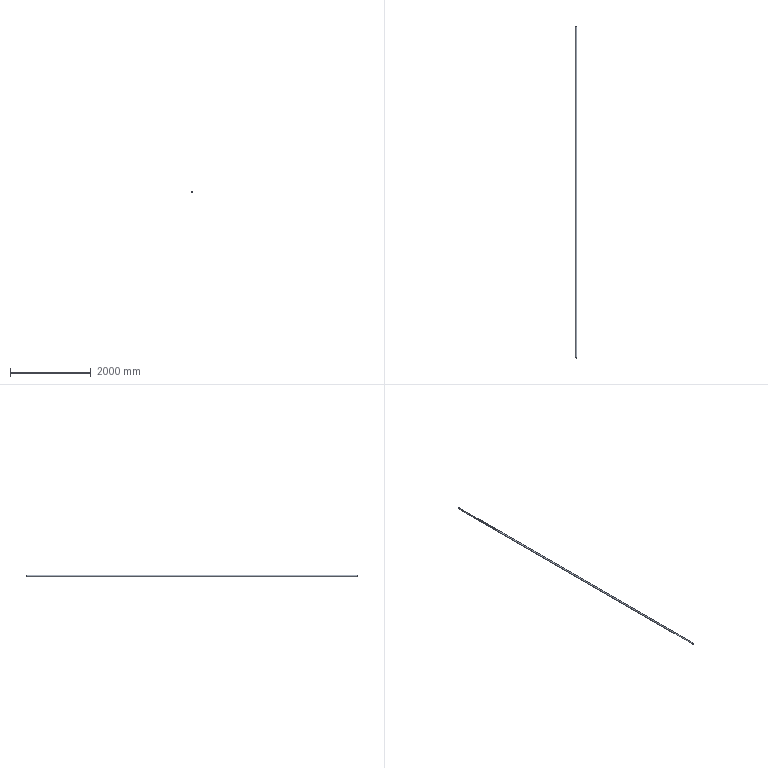Component | NX | 43_8 | 1 solid | 4 faces | volume 2756700 mm3 | cylinder 2 | plane 2 | commonest cylinder face diameters 34 x1 27 x1